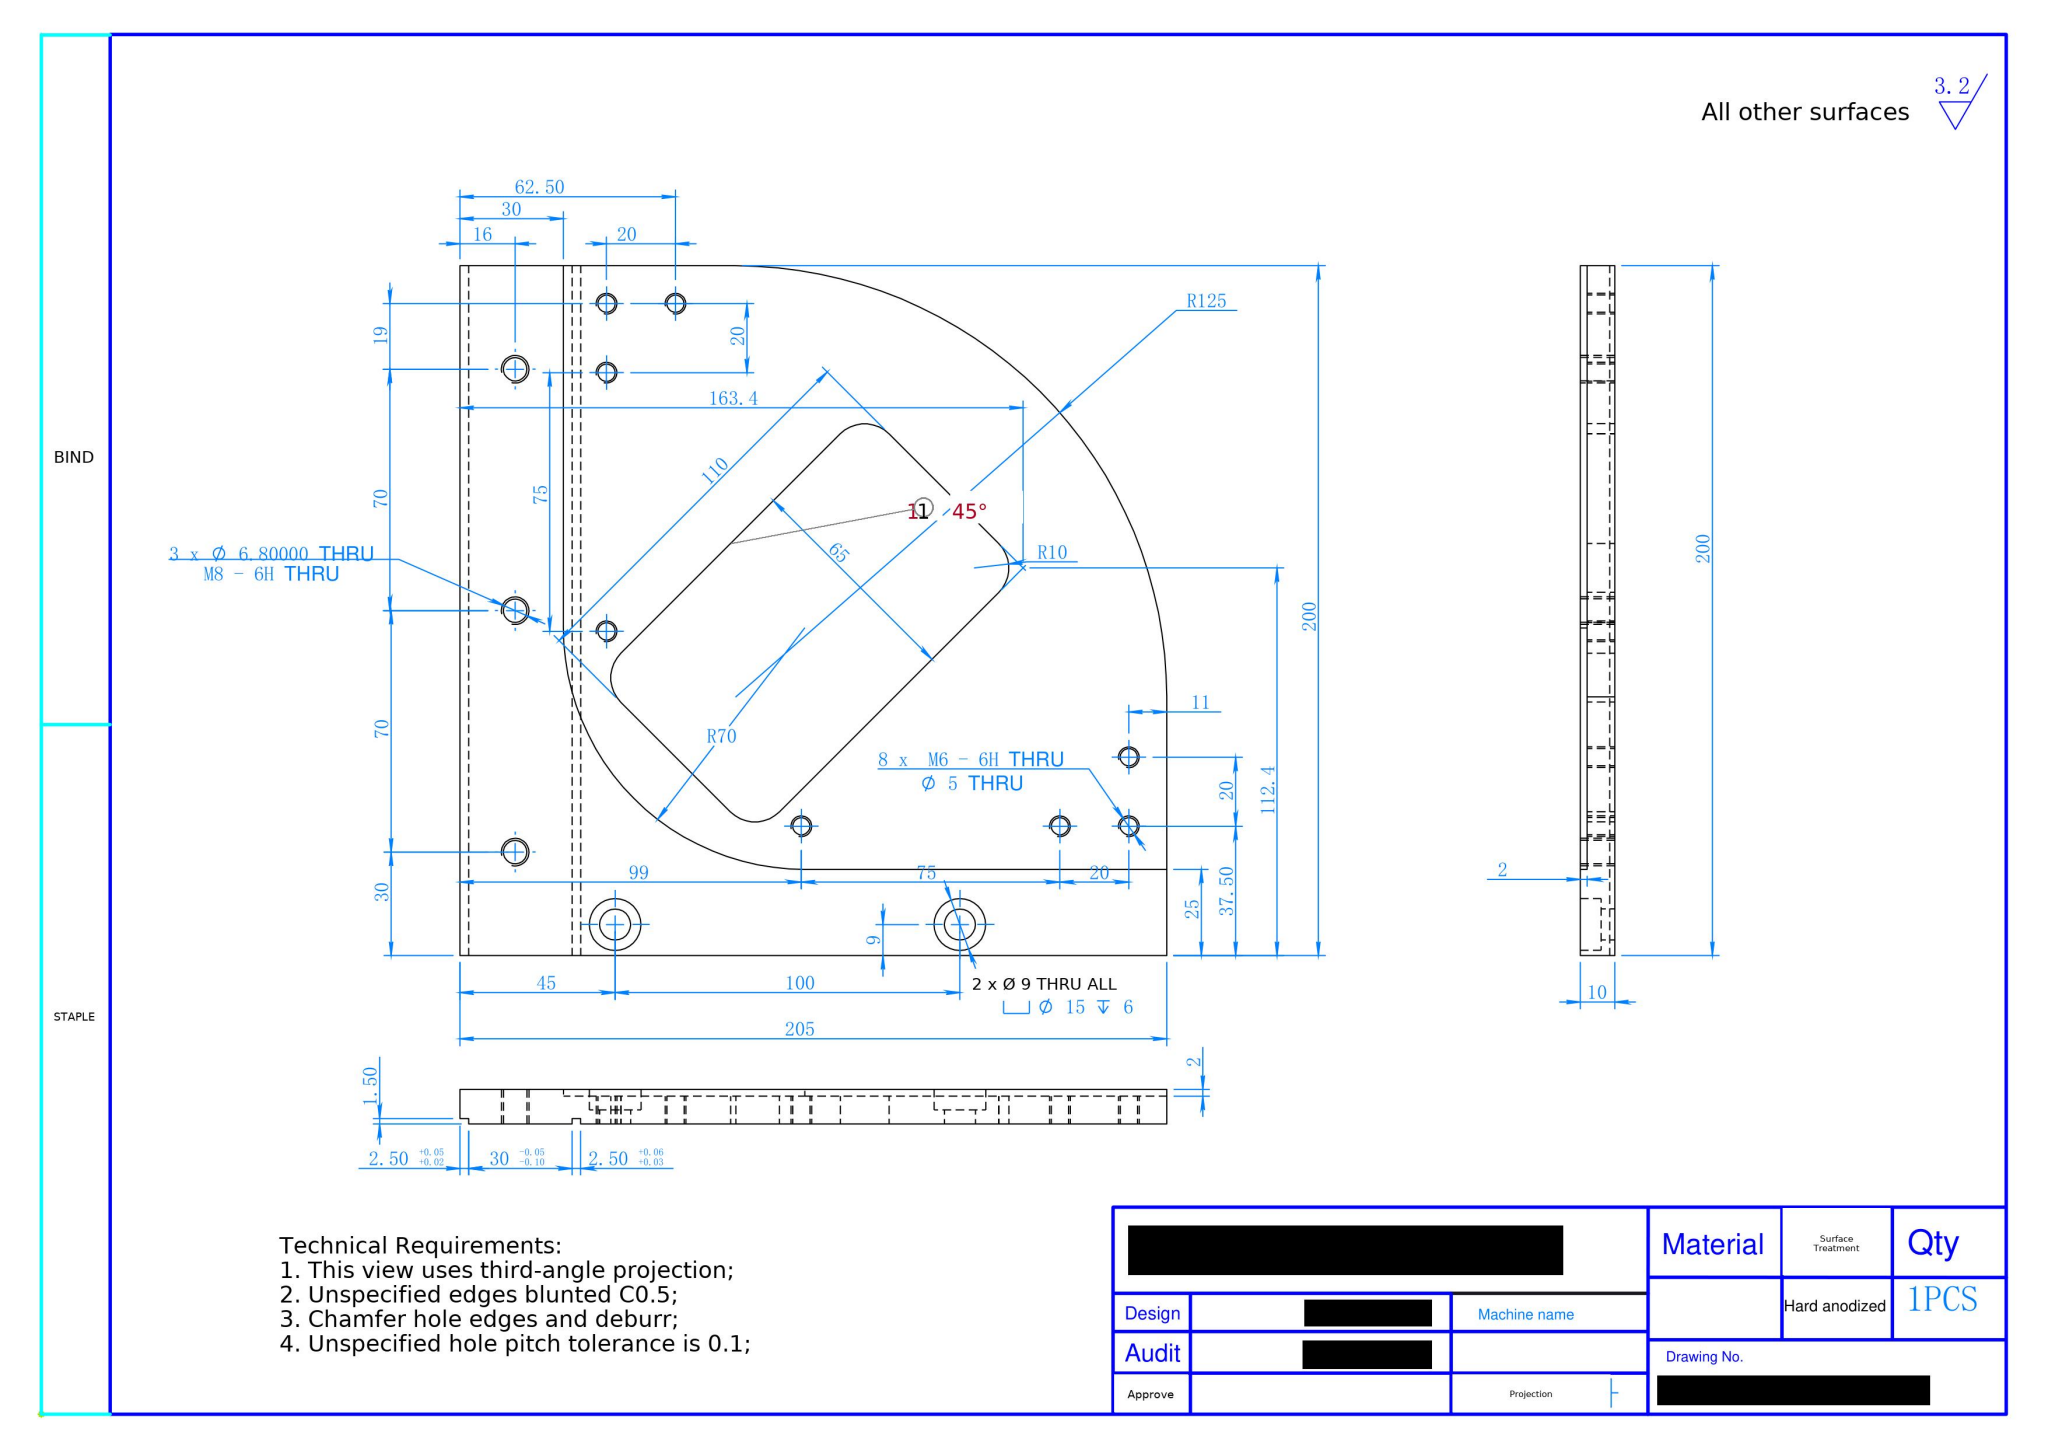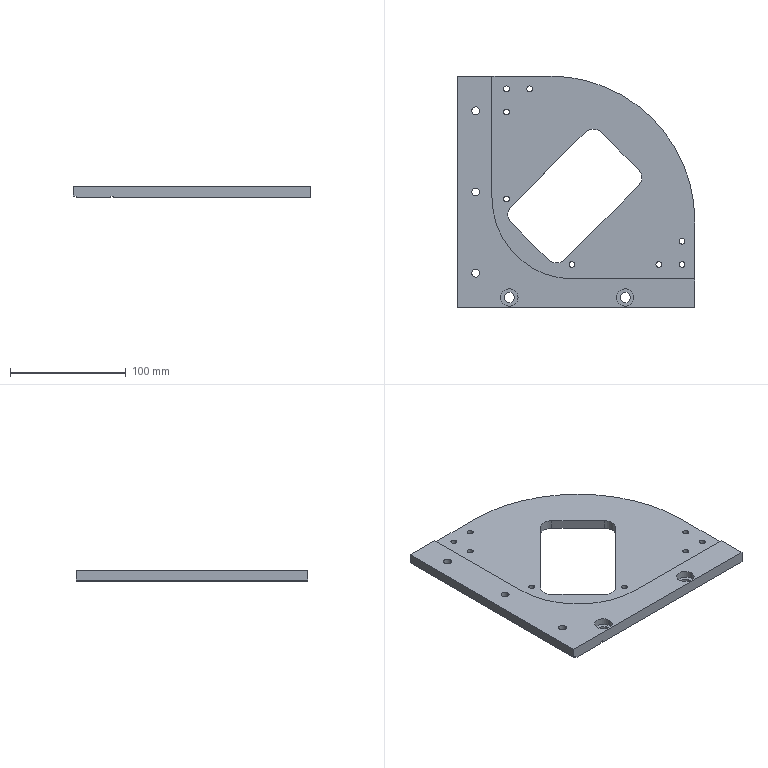Part | SolidWorks | mm | 1 solid | 57 faces | box 205 x 200 x 10 mm | volume 261039 mm3 | cylinder 36 | plane 21 | commonest cylinder face diameters 5 x16 6.8 x6 15 x4 9 x4 20 x4 250 x1 140 x1
build123d program:
from build123d import *

# Parameters (mm, degrees)
BOSS_EXTRUDE1_DEPTH                               = 10
SKETCH2_W                                         = 175
SKETCH2_H                                         = 175
CUT_EXTRUDE1_DEPTH                                = 2
FILLET1_R                                         = 70
FILLET2_R                                         = 10
MOVE_FACE2_BY                                     = 5
SKETCH10_W                                        = 3
SKETCH10_H                                        = 3
SKETCH10_W_2                                      = 2.5
CUT_EXTRUDE7_DEPTH                                = 392
HOLE_SIZE_ACCORDING_TO_TYPE_OF_HEXAGO_D           = 9
HOLE_SIZE_ACCORDING_TO_TYPE_OF_HEXAGO_CBORE_D     = 15
HOLE_SIZE_ACCORDING_TO_TYPE_OF_HEXAGO_CBORE_DEPTH = 6
M6_TAPPED_HOLE1_D                                 = 5
M8_TAPPED_HOLE1_D                                 = 6.8


with BuildPart() as part:
    # Sketch1 → Boss-Extrude1 (new body)
    with BuildSketch(Plane.XY):
        with BuildLine():
            Line((-25, 100), (-100, 100))
            Line((-100, 100), (-100, -100))
            Line((-100, -100), (100, -100))
            Line((100, -100), (100, -25))
            ThreePointArc((100, -25), (63.388, 63.388), (-25, 100))
        make_face()
        Polygon((12.374, 58.336), (58.336, 12.374), (-19.445, -65.407), (-65.407, -19.445), align=None, mode=Mode.SUBTRACT)
    extrude(amount=BOSS_EXTRUDE1_DEPTH)

    # Sketch2 → Cut-Extrude1 (cut)
    with BuildSketch(Plane.XY.offset(10)):
        with Locations((12.5, 12.5)):
            Rectangle(SKETCH2_W, SKETCH2_H)
    extrude(amount=-CUT_EXTRUDE1_DEPTH, mode=Mode.SUBTRACT)

    # Fillet1
    fillet1_edges = [part.edges().sort_by_distance(p)[0] for p in [
        (-75, -75, 9),
    ]]
    fillet(fillet1_edges, radius=FILLET1_R)

    # Fillet2
    fillet2_edges = [part.edges().sort_by_distance(p)[0] for p in [
        (12.374, 58.336, 4),
        (-65.407, -19.445, 4),
        (-19.445, -65.407, 4),
        (58.336, 12.374, 4),
    ]]
    fillet(fillet2_edges, radius=FILLET2_R)

    # Move Face2: a face moved outward by 5.0
    extrude(part.faces().sort_by_distance((-100, 0, 5))[0], amount=MOVE_FACE2_BY, dir=(-1, 0, 0))

    # Sketch10 → Cut-Extrude7 (cut)
    with BuildSketch(Plane(origin=(0, 100, 0), x_dir=(1, 0, 0), z_dir=(0, 1, 0))):
        with Locations((-104, 0)):
            Rectangle(SKETCH10_W, SKETCH10_H)
        with Locations((-71.25, 0)):
            Rectangle(SKETCH10_W_2, SKETCH10_H)
    extrude(amount=-CUT_EXTRUDE7_DEPTH, mode=Mode.SUBTRACT)

    # Hole Size _ according to_ type of Hexago (through all)
    with Locations(Plane.XY.offset(10)):
        with Locations((40, -91), (-60, -91)):
            CounterBoreHole(HOLE_SIZE_ACCORDING_TO_TYPE_OF_HEXAGO_D / 2, HOLE_SIZE_ACCORDING_TO_TYPE_OF_HEXAGO_CBORE_D / 2, HOLE_SIZE_ACCORDING_TO_TYPE_OF_HEXAGO_CBORE_DEPTH)

    # M6 Tapped Hole1 (through all)
    with Locations(Plane.XY.offset(8)):
        with Locations((89, -62.5), (69, -62.5), (89, -42.5), (-6, -62.5), (-62.5, -6), (-62.5, 89), (-62.5, 69), (-42.5, 89)):
            Hole(M6_TAPPED_HOLE1_D / 2)

    # M8 Tapped Hole1 (through all)
    with Locations(Plane.XY.offset(10)):
        with Locations((-89, 70), (-89, 0), (-89, -70)):
            Hole(M8_TAPPED_HOLE1_D / 2)


solid = part.part